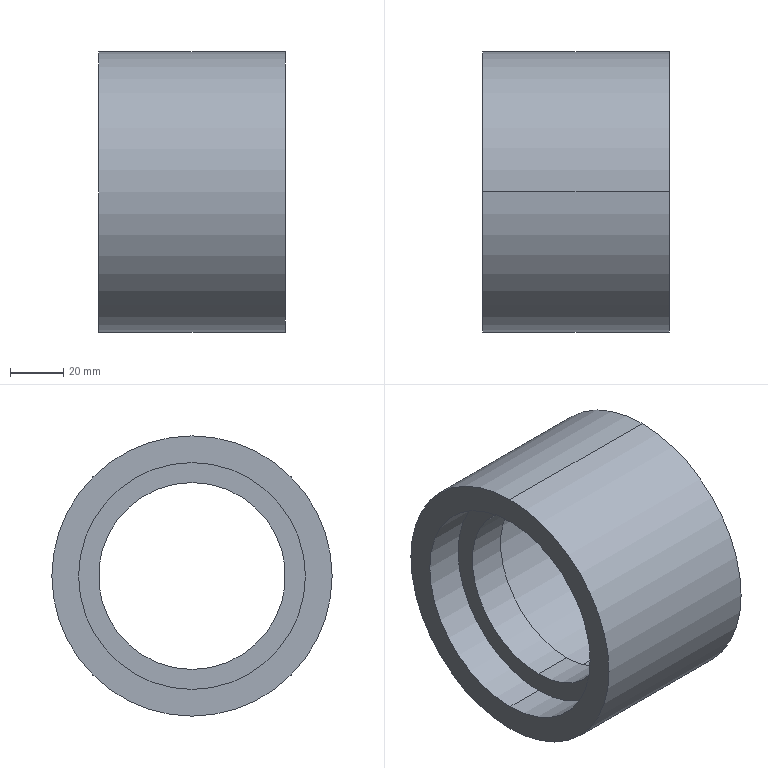Component | SolidWorks | bearing dan rumahan assembly-1_rumah bearing-1 | 1 solid | 24 faces | box 70 x 105 x 105 mm | volume 234610 mm3 | cylinder 16 | plane 8 | commonest cylinder face diameters 6 x8 85 x4 70 x2 105 x2 | material ASTM A36 Steel
build123d program:
from build123d import *

# Parameters (mm, degrees)
BOSS_EXTRUDE1_DEPTH      = 40
BOSS_EXTRUDE1_DEPTH_BACK = 30
SKETCH1_R                = 52.5
SKETCH1_R_2              = 42.5
SKETCH2_R                = 42.5
SKETCH2_R_2              = 35
BOSS_EXTRUDE2_DEPTH      = 15
SKETCH3_R                = 3
CUT_EXTRUDE1_DEPTH       = 15


with BuildPart() as part:
    # Sketch1 → Boss-Extrude1 (new, two sides: drawn at the far end of the back side and taken through both)
    with BuildSketch(Plane(origin=(0, 0, 0), x_dir=(0, 0, -1), z_dir=(1, 0, 0)).offset(-BOSS_EXTRUDE1_DEPTH_BACK)):
        Circle(SKETCH1_R)
        Circle(SKETCH1_R_2, mode=Mode.SUBTRACT)
    extrude(amount=BOSS_EXTRUDE1_DEPTH + BOSS_EXTRUDE1_DEPTH_BACK)

    # Sketch2 → Boss-Extrude2 (add)
    with BuildSketch(Plane(origin=(0, 0, 0), x_dir=(0, 0, -1), z_dir=(1, 0, 0))):
        Circle(SKETCH2_R)
        Circle(SKETCH2_R_2, mode=Mode.SUBTRACT)
    extrude(amount=-BOSS_EXTRUDE2_DEPTH)

    # Sketch3 → Cut-Extrude1 (cut)
    with BuildSketch(Plane(origin=(40, 0, 0), x_dir=(0, 0, -1), z_dir=(1, 0, 0))):
        with Locations((0, 47.5)):
            Circle(SKETCH3_R)
        with Locations((47.5, 0)):
            Circle(SKETCH3_R)
        with Locations((0, -47.5)):
            Circle(SKETCH3_R)
        with Locations((-47.5, 0)):
            Circle(SKETCH3_R)
    extrude(amount=-CUT_EXTRUDE1_DEPTH, mode=Mode.SUBTRACT)


solid = part.part

# Placed as in the assembly
solid = solid.moved(Location((-2.5, -110, 40), (0, 0, 0)))
STEP:
#1=COLOUR_RGB('',0.7922,0.8196,0.9333);
#2=FILL_AREA_STYLE_COLOUR('',#1);
#3=FILL_AREA_STYLE('',(#2));
#4=SURFACE_STYLE_FILL_AREA(#3);
#5=SURFACE_SIDE_STYLE('',(#4));
#6=SURFACE_STYLE_USAGE(.BOTH.,#5);
#7=PRESENTATION_STYLE_ASSIGNMENT((#6));
#8=CARTESIAN_POINT('',(0.8858,-2.461,1.693));
#9=VERTEX_POINT('',#8);
#10=CARTESIAN_POINT('',(0.8858,-2.461,1.457));
#11=VERTEX_POINT('',#10);
#12=CARTESIAN_POINT('',(0.8858,-2.461,1.575));
#13=DIRECTION('',(1.,-0.,-0.));
#14=DIRECTION('',(0.,0.,-1.));
#15=AXIS2_PLACEMENT_3D('',#12,#13,#14);
#16=CIRCLE('',#15,0.1181);
#17=EDGE_CURVE('',#9,#11,#16,.T.);
#18=ORIENTED_EDGE('',*,*,#17,.F.);
#19=CARTESIAN_POINT('',(1.476,-2.461,1.693));
#20=VERTEX_POINT('',#19);
#21=CARTESIAN_POINT('',(0.8858,-2.461,1.693));
#22=DIRECTION('',(1.,-0.,-0.));
#23=VECTOR('',#22,39.37);
#24=LINE('',#21,#23);
#25=EDGE_CURVE('',#9,#20,#24,.T.);
#26=ORIENTED_EDGE('',*,*,#25,.T.);
#27=CARTESIAN_POINT('',(1.476,-2.461,1.457));
#28=VERTEX_POINT('',#27);
#29=CARTESIAN_POINT('',(1.476,-2.461,1.575));
#30=DIRECTION('',(1.,-0.,-0.));
#31=DIRECTION('',(0.,0.,-1.));
#32=AXIS2_PLACEMENT_3D('',#29,#30,#31);
#33=CIRCLE('',#32,0.1181);
#34=EDGE_CURVE('',#20,#28,#33,.T.);
#35=ORIENTED_EDGE('',*,*,#34,.T.);
#36=CARTESIAN_POINT('',(0.8858,-2.461,1.457));
#37=DIRECTION('',(1.,-0.,-0.));
#38=VECTOR('',#37,39.37);
#39=LINE('',#36,#38);
#40=EDGE_CURVE('',#11,#28,#39,.T.);
#41=ORIENTED_EDGE('',*,*,#40,.F.);
#42=EDGE_LOOP('',(#18,#26,#35,#41));
#43=FACE_OUTER_BOUND('',#42,.T.);
#44=CARTESIAN_POINT('',(0.8858,-2.461,1.575));
#45=DIRECTION('',(1.,-0.,-0.));
#46=DIRECTION('',(0.,0.,-1.));
#47=AXIS2_PLACEMENT_3D('',#44,#45,#46);
#48=CYLINDRICAL_SURFACE('',#47,0.1181);
#49=ADVANCED_FACE('',(#43),#48,.F.);
#50=CARTESIAN_POINT('',(0.8858,-4.331,-0.1772));
#51=VERTEX_POINT('',#50);
#52=CARTESIAN_POINT('',(0.8858,-4.331,-0.4134));
#53=VERTEX_POINT('',#52);
#54=CARTESIAN_POINT('',(0.8858,-4.331,-0.2953));
#55=DIRECTION('',(1.,-0.,-0.));
#56=DIRECTION('',(0.,0.,-1.));
#57=AXIS2_PLACEMENT_3D('',#54,#55,#56);
#58=CIRCLE('',#57,0.1181);
#59=EDGE_CURVE('',#51,#53,#58,.T.);
#60=ORIENTED_EDGE('',*,*,#59,.F.);
#61=CARTESIAN_POINT('',(1.476,-4.331,-0.1772));
#62=VERTEX_POINT('',#61);
#63=CARTESIAN_POINT('',(0.8858,-4.331,-0.1772));
#64=DIRECTION('',(1.,-0.,-0.));
#65=VECTOR('',#64,39.37);
#66=LINE('',#63,#65);
#67=EDGE_CURVE('',#51,#62,#66,.T.);
#68=ORIENTED_EDGE('',*,*,#67,.T.);
#69=CARTESIAN_POINT('',(1.476,-4.331,-0.4134));
#70=VERTEX_POINT('',#69);
#71=CARTESIAN_POINT('',(1.476,-4.331,-0.2953));
#72=DIRECTION('',(1.,-0.,-0.));
#73=DIRECTION('',(0.,0.,-1.));
#74=AXIS2_PLACEMENT_3D('',#71,#72,#73);
#75=CIRCLE('',#74,0.1181);
#76=EDGE_CURVE('',#62,#70,#75,.T.);
#77=ORIENTED_EDGE('',*,*,#76,.T.);
#78=CARTESIAN_POINT('',(0.8858,-4.331,-0.4134));
#79=DIRECTION('',(1.,-0.,-0.));
#80=VECTOR('',#79,39.37);
#81=LINE('',#78,#80);
#82=EDGE_CURVE('',#53,#70,#81,.T.);
#83=ORIENTED_EDGE('',*,*,#82,.F.);
#84=EDGE_LOOP('',(#60,#68,#77,#83));
#85=FACE_OUTER_BOUND('',#84,.T.);
#86=CARTESIAN_POINT('',(0.8858,-4.331,-0.2953));
#87=DIRECTION('',(1.,-0.,-0.));
#88=DIRECTION('',(0.,0.,-1.));
#89=AXIS2_PLACEMENT_3D('',#86,#87,#88);
#90=CYLINDRICAL_SURFACE('',#89,0.1181);
#91=ADVANCED_FACE('',(#85),#90,.F.);
#92=CARTESIAN_POINT('',(0.8858,-6.201,1.693));
#93=VERTEX_POINT('',#92);
#94=CARTESIAN_POINT('',(0.8858,-6.201,1.457));
#95=VERTEX_POINT('',#94);
#96=CARTESIAN_POINT('',(0.8858,-6.201,1.575));
#97=DIRECTION('',(1.,-0.,-0.));
#98=DIRECTION('',(0.,0.,-1.));
#99=AXIS2_PLACEMENT_3D('',#96,#97,#98);
#100=CIRCLE('',#99,0.1181);
#101=EDGE_CURVE('',#93,#95,#100,.T.);
#102=ORIENTED_EDGE('',*,*,#101,.F.);
#103=CARTESIAN_POINT('',(1.476,-6.201,1.693));
#104=VERTEX_POINT('',#103);
#105=CARTESIAN_POINT('',(0.8858,-6.201,1.693));
#106=DIRECTION('',(1.,-0.,-0.));
#107=VECTOR('',#106,39.37);
#108=LINE('',#105,#107);
#109=EDGE_CURVE('',#93,#104,#108,.T.);
#110=ORIENTED_EDGE('',*,*,#109,.T.);
#111=CARTESIAN_POINT('',(1.476,-6.201,1.457));
#112=VERTEX_POINT('',#111);
#113=CARTESIAN_POINT('',(1.476,-6.201,1.575));
#114=DIRECTION('',(1.,-0.,-0.));
#115=DIRECTION('',(0.,0.,-1.));
#116=AXIS2_PLACEMENT_3D('',#113,#114,#115);
#117=CIRCLE('',#116,0.1181);
#118=EDGE_CURVE('',#104,#112,#117,.T.);
#119=ORIENTED_EDGE('',*,*,#118,.T.);
#120=CARTESIAN_POINT('',(0.8858,-6.201,1.457));
#121=DIRECTION('',(1.,-0.,-0.));
#122=VECTOR('',#121,39.37);
#123=LINE('',#120,#122);
#124=EDGE_CURVE('',#95,#112,#123,.T.);
#125=ORIENTED_EDGE('',*,*,#124,.F.);
#126=EDGE_LOOP('',(#102,#110,#119,#125));
#127=FACE_OUTER_BOUND('',#126,.T.);
#128=CARTESIAN_POINT('',(0.8858,-6.201,1.575));
#129=DIRECTION('',(1.,-0.,-0.));
#130=DIRECTION('',(0.,0.,-1.));
#131=AXIS2_PLACEMENT_3D('',#128,#129,#130);
#132=CYLINDRICAL_SURFACE('',#131,0.1181);
#133=ADVANCED_FACE('',(#127),#132,.F.);
#134=CARTESIAN_POINT('',(0.8858,-4.331,3.563));
#135=VERTEX_POINT('',#134);
#136=CARTESIAN_POINT('',(0.8858,-4.331,3.327));
#137=VERTEX_POINT('',#136);
#138=CARTESIAN_POINT('',(0.8858,-4.331,3.445));
#139=DIRECTION('',(1.,-0.,-0.));
#140=DIRECTION('',(0.,0.,-1.));
#141=AXIS2_PLACEMENT_3D('',#138,#139,#140);
#142=CIRCLE('',#141,0.1181);
#143=EDGE_CURVE('',#135,#137,#142,.T.);
#144=ORIENTED_EDGE('',*,*,#143,.F.);
#145=CARTESIAN_POINT('',(1.476,-4.331,3.563));
#146=VERTEX_POINT('',#145);
#147=CARTESIAN_POINT('',(0.8858,-4.331,3.563));
#148=DIRECTION('',(1.,-0.,-0.));
#149=VECTOR('',#148,39.37);
#150=LINE('',#147,#149);
#151=EDGE_CURVE('',#135,#146,#150,.T.);
#152=ORIENTED_EDGE('',*,*,#151,.T.);
#153=CARTESIAN_POINT('',(1.476,-4.331,3.327));
#154=VERTEX_POINT('',#153);
#155=CARTESIAN_POINT('',(1.476,-4.331,3.445));
#156=DIRECTION('',(1.,-0.,-0.));
#157=DIRECTION('',(0.,0.,-1.));
#158=AXIS2_PLACEMENT_3D('',#155,#156,#157);
#159=CIRCLE('',#158,0.1181);
#160=EDGE_CURVE('',#146,#154,#159,.T.);
#161=ORIENTED_EDGE('',*,*,#160,.T.);
#162=CARTESIAN_POINT('',(0.8858,-4.331,3.327));
#163=DIRECTION('',(1.,-0.,-0.));
#164=VECTOR('',#163,39.37);
#165=LINE('',#162,#164);
#166=EDGE_CURVE('',#137,#154,#165,.T.);
#167=ORIENTED_EDGE('',*,*,#166,.F.);
#168=EDGE_LOOP('',(#144,#152,#161,#167));
#169=FACE_OUTER_BOUND('',#168,.T.);
#170=CARTESIAN_POINT('',(0.8858,-4.331,3.445));
#171=DIRECTION('',(1.,-0.,-0.));
#172=DIRECTION('',(0.,0.,-1.));
#173=AXIS2_PLACEMENT_3D('',#170,#171,#172);
#174=CYLINDRICAL_SURFACE('',#173,0.1181);
#175=ADVANCED_FACE('',(#169),#174,.F.);
#176=CARTESIAN_POINT('',(-0.689,-4.331,2.953));
#177=VERTEX_POINT('',#176);
#178=CARTESIAN_POINT('',(-0.689,-4.331,0.1969));
#179=VERTEX_POINT('',#178);
#180=CARTESIAN_POINT('',(-0.689,-4.331,1.575));
#181=DIRECTION('',(1.,-0.,-0.));
#182=DIRECTION('',(-0.,0.,-1.));
#183=AXIS2_PLACEMENT_3D('',#180,#181,#182);
#184=CIRCLE('',#183,1.378);
#185=EDGE_CURVE('',#177,#179,#184,.T.);
#186=ORIENTED_EDGE('',*,*,#185,.F.);
#187=CARTESIAN_POINT('',(-0.09843,-4.331,2.953));
#188=VERTEX_POINT('',#187);
#189=CARTESIAN_POINT('',(-0.689,-4.331,2.953));
#190=DIRECTION('',(1.,-0.,-0.));
#191=VECTOR('',#190,39.37);
#192=LINE('',#189,#191);
#193=EDGE_CURVE('',#177,#188,#192,.T.);
#194=ORIENTED_EDGE('',*,*,#193,.T.);
#195=CARTESIAN_POINT('',(-0.09843,-4.331,0.1969));
#196=VERTEX_POINT('',#195);
#197=CARTESIAN_POINT('',(-0.09843,-4.331,1.575));
#198=DIRECTION('',(1.,-0.,-0.));
#199=DIRECTION('',(-0.,0.,-1.));
#200=AXIS2_PLACEMENT_3D('',#197,#198,#199);
#201=CIRCLE('',#200,1.378);
#202=EDGE_CURVE('',#188,#196,#201,.T.);
#203=ORIENTED_EDGE('',*,*,#202,.T.);
#204=CARTESIAN_POINT('',(-0.689,-4.331,0.1969));
#205=DIRECTION('',(1.,-0.,-0.));
#206=VECTOR('',#205,39.37);
#207=LINE('',#204,#206);
#208=EDGE_CURVE('',#179,#196,#207,.T.);
#209=ORIENTED_EDGE('',*,*,#208,.F.);
#210=EDGE_LOOP('',(#186,#194,#203,#209));
#211=FACE_OUTER_BOUND('',#210,.T.);
#212=CARTESIAN_POINT('',(-0.689,-4.331,1.575));
#213=DIRECTION('',(1.,-0.,-0.));
#214=DIRECTION('',(-0.,0.,-1.));
#215=AXIS2_PLACEMENT_3D('',#212,#213,#214);
#216=CYLINDRICAL_SURFACE('',#215,1.378);
#217=ADVANCED_FACE('',(#211),#216,.F.);
#218=CARTESIAN_POINT('',(-0.09843,-4.331,3.248));
#219=VERTEX_POINT('',#218);
#220=CARTESIAN_POINT('',(-0.09843,-4.331,-0.09843));
#221=VERTEX_POINT('',#220);
#222=CARTESIAN_POINT('',(-0.09843,-4.331,1.575));
#223=DIRECTION('',(1.,-0.,-0.));
#224=DIRECTION('',(-0.,0.,-1.));
#225=AXIS2_PLACEMENT_3D('',#222,#223,#224);
#226=CIRCLE('',#225,1.673);
#227=EDGE_CURVE('',#219,#221,#226,.T.);
#228=ORIENTED_EDGE('',*,*,#227,.F.);
#229=CARTESIAN_POINT('',(1.476,-4.331,3.248));
#230=VERTEX_POINT('',#229);
#231=CARTESIAN_POINT('',(-1.28,-4.331,3.248));
#232=DIRECTION('',(1.,-0.,-0.));
#233=VECTOR('',#232,39.37);
#234=LINE('',#231,#233);
#235=EDGE_CURVE('',#219,#230,#234,.T.);
#236=ORIENTED_EDGE('',*,*,#235,.T.);
#237=CARTESIAN_POINT('',(1.476,-4.331,-0.09843));
#238=VERTEX_POINT('',#237);
#239=CARTESIAN_POINT('',(1.476,-4.331,1.575));
#240=DIRECTION('',(1.,-0.,-0.));
#241=DIRECTION('',(-0.,0.,-1.));
#242=AXIS2_PLACEMENT_3D('',#239,#240,#241);
#243=CIRCLE('',#242,1.673);
#244=EDGE_CURVE('',#230,#238,#243,.T.);
#245=ORIENTED_EDGE('',*,*,#244,.T.);
#246=CARTESIAN_POINT('',(-1.28,-4.331,-0.09843));
#247=DIRECTION('',(1.,-0.,-0.));
#248=VECTOR('',#247,39.37);
#249=LINE('',#246,#248);
#250=EDGE_CURVE('',#221,#238,#249,.T.);
#251=ORIENTED_EDGE('',*,*,#250,.F.);
#252=EDGE_LOOP('',(#228,#236,#245,#251));
#253=FACE_OUTER_BOUND('',#252,.T.);
#254=CARTESIAN_POINT('',(-1.28,-4.331,1.575));
#255=DIRECTION('',(1.,-0.,-0.));
#256=DIRECTION('',(-0.,0.,-1.));
#257=AXIS2_PLACEMENT_3D('',#254,#255,#256);
#258=CYLINDRICAL_SURFACE('',#257,1.673);
#259=ADVANCED_FACE('',(#253),#258,.F.);
#260=CARTESIAN_POINT('',(-1.28,-4.331,-0.4921));
#261=VERTEX_POINT('',#260);
#262=CARTESIAN_POINT('',(-1.28,-4.331,3.642));
#263=VERTEX_POINT('',#262);
#264=CARTESIAN_POINT('',(-1.28,-4.331,1.575));
#265=DIRECTION('',(1.,-0.,-0.));
#266=DIRECTION('',(-0.,0.,-1.));
#267=AXIS2_PLACEMENT_3D('',#264,#265,#266);
#268=CIRCLE('',#267,2.067);
#269=EDGE_CURVE('',#261,#263,#268,.T.);
#270=ORIENTED_EDGE('',*,*,#269,.T.);
#271=CARTESIAN_POINT('',(1.476,-4.331,3.642));
#272=VERTEX_POINT('',#271);
#273=CARTESIAN_POINT('',(-1.28,-4.331,3.642));
#274=DIRECTION('',(1.,-0.,-0.));
#275=VECTOR('',#274,39.37);
#276=LINE('',#273,#275);
#277=EDGE_CURVE('',#263,#272,#276,.T.);
#278=ORIENTED_EDGE('',*,*,#277,.T.);
#279=CARTESIAN_POINT('',(1.476,-4.331,-0.4921));
#280=VERTEX_POINT('',#279);
#281=CARTESIAN_POINT('',(1.476,-4.331,1.575));
#282=DIRECTION('',(1.,-0.,-0.));
#283=DIRECTION('',(-0.,0.,-1.));
#284=AXIS2_PLACEMENT_3D('',#281,#282,#283);
#285=CIRCLE('',#284,2.067);
#286=EDGE_CURVE('',#280,#272,#285,.T.);
#287=ORIENTED_EDGE('',*,*,#286,.F.);
#288=CARTESIAN_POINT('',(-1.28,-4.331,-0.4921));
#289=DIRECTION('',(1.,-0.,-0.));
#290=VECTOR('',#289,39.37);
#291=LINE('',#288,#290);
#292=EDGE_CURVE('',#261,#280,#291,.T.);
#293=ORIENTED_EDGE('',*,*,#292,.F.);
#294=EDGE_LOOP('',(#270,#278,#287,#293));
#295=FACE_OUTER_BOUND('',#294,.T.);
#296=CARTESIAN_POINT('',(-1.28,-4.331,1.575));
#297=DIRECTION('',(1.,-0.,-0.));
#298=DIRECTION('',(-0.,0.,-1.));
#299=AXIS2_PLACEMENT_3D('',#296,#297,#298);
#300=CYLINDRICAL_SURFACE('',#299,2.067);
#301=ADVANCED_FACE('',(#295),#300,.T.);
#302=CARTESIAN_POINT('',(-1.28,-4.331,3.248));
#303=VERTEX_POINT('',#302);
#304=CARTESIAN_POINT('',(-1.28,-4.331,-0.09843));
#305=VERTEX_POINT('',#304);
#306=CARTESIAN_POINT('',(-1.28,-4.331,1.575));
#307=DIRECTION('',(1.,-0.,-0.));
#308=DIRECTION('',(-0.,0.,-1.));
#309=AXIS2_PLACEMENT_3D('',#306,#307,#308);
#310=CIRCLE('',#309,1.673);
#311=EDGE_CURVE('',#303,#305,#310,.T.);
#312=ORIENTED_EDGE('',*,*,#311,.F.);
#313=CARTESIAN_POINT('',(-0.689,-4.331,3.248));
#314=VERTEX_POINT('',#313);
#315=CARTESIAN_POINT('',(-1.28,-4.331,3.248));
#316=DIRECTION('',(1.,-0.,-0.));
#317=VECTOR('',#316,39.37);
#318=LINE('',#315,#317);
#319=EDGE_CURVE('',#303,#314,#318,.T.);
#320=ORIENTED_EDGE('',*,*,#319,.T.);
#321=CARTESIAN_POINT('',(-0.689,-4.331,-0.09843));
#322=VERTEX_POINT('',#321);
#323=CARTESIAN_POINT('',(-0.689,-4.331,1.575));
#324=DIRECTION('',(-1.,0.,0.));
#325=DIRECTION('',(-0.,0.,-1.));
#326=AXIS2_PLACEMENT_3D('',#323,#324,#325);
#327=CIRCLE('',#326,1.673);
#328=EDGE_CURVE('',#322,#314,#327,.T.);
#329=ORIENTED_EDGE('',*,*,#328,.F.);
#330=CARTESIAN_POINT('',(-1.28,-4.331,-0.09843));
#331=DIRECTION('',(1.,-0.,-0.));
#332=VECTOR('',#331,39.37);
#333=LINE('',#330,#332);
#334=EDGE_CURVE('',#305,#322,#333,.T.);
#335=ORIENTED_EDGE('',*,*,#334,.F.);
#336=EDGE_LOOP('',(#312,#320,#329,#335));
#337=FACE_OUTER_BOUND('',#336,.T.);
#338=CARTESIAN_POINT('',(-1.28,-4.331,1.575));
#339=DIRECTION('',(1.,-0.,-0.));
#340=DIRECTION('',(-0.,0.,-1.));
#341=AXIS2_PLACEMENT_3D('',#338,#339,#340);
#342=CYLINDRICAL_SURFACE('',#341,1.673);
#343=ADVANCED_FACE('',(#337),#342,.F.);
#344=ORIENTED_EDGE('',*,*,#319,.F.);
#345=CARTESIAN_POINT('',(-1.28,-4.331,1.575));
#346=DIRECTION('',(1.,-0.,-0.));
#347=DIRECTION('',(-0.,0.,-1.));
#348=AXIS2_PLACEMENT_3D('',#345,#346,#347);
#349=CIRCLE('',#348,1.673);
#350=EDGE_CURVE('',#305,#303,#349,.T.);
#351=ORIENTED_EDGE('',*,*,#350,.F.);
#352=ORIENTED_EDGE('',*,*,#334,.T.);
#353=CARTESIAN_POINT('',(-0.689,-4.331,1.575));
#354=DIRECTION('',(-1.,0.,0.));
#355=DIRECTION('',(-0.,0.,-1.));
#356=AXIS2_PLACEMENT_3D('',#353,#354,#355);
#357=CIRCLE('',#356,1.673);
#358=EDGE_CURVE('',#314,#322,#357,.T.);
#359=ORIENTED_EDGE('',*,*,#358,.F.);
#360=EDGE_LOOP('',(#344,#351,#352,#359));
#361=FACE_OUTER_BOUND('',#360,.T.);
#362=CARTESIAN_POINT('',(-1.28,-4.331,1.575));
#363=DIRECTION('',(1.,-0.,-0.));
#364=DIRECTION('',(-0.,0.,-1.));
#365=AXIS2_PLACEMENT_3D('',#362,#363,#364);
#366=CYLINDRICAL_SURFACE('',#365,1.673);
#367=ADVANCED_FACE('',(#361),#366,.F.);
#368=ORIENTED_EDGE('',*,*,#277,.F.);
#369=CARTESIAN_POINT('',(-1.28,-4.331,1.575));
#370=DIRECTION('',(1.,-0.,-0.));
#371=DIRECTION('',(-0.,0.,-1.));
#372=AXIS2_PLACEMENT_3D('',#369,#370,#371);
#373=CIRCLE('',#372,2.067);
#374=EDGE_CURVE('',#263,#261,#373,.T.);
#375=ORIENTED_EDGE('',*,*,#374,.T.);
#376=ORIENTED_EDGE('',*,*,#292,.T.);
#377=CARTESIAN_POINT('',(1.476,-4.331,1.575));
#378=DIRECTION('',(1.,-0.,-0.));
#379=DIRECTION('',(-0.,0.,-1.));
#380=AXIS2_PLACEMENT_3D('',#377,#378,#379);
#381=CIRCLE('',#380,2.067);
#382=EDGE_CURVE('',#272,#280,#381,.T.);
#383=ORIENTED_EDGE('',*,*,#382,.F.);
#384=EDGE_LOOP('',(#368,#375,#376,#383));
#385=FACE_OUTER_BOUND('',#384,.T.);
#386=CARTESIAN_POINT('',(-1.28,-4.331,1.575));
#387=DIRECTION('',(1.,-0.,-0.));
#388=DIRECTION('',(-0.,0.,-1.));
#389=AXIS2_PLACEMENT_3D('',#386,#387,#388);
#390=CYLINDRICAL_SURFACE('',#389,2.067);
#391=ADVANCED_FACE('',(#385),#390,.T.);
#392=ORIENTED_EDGE('',*,*,#350,.T.);
#393=ORIENTED_EDGE('',*,*,#311,.T.);
#394=EDGE_LOOP('',(#392,#393));
#395=FACE_BOUND('',#394,.T.);
#396=ORIENTED_EDGE('',*,*,#269,.F.);
#397=ORIENTED_EDGE('',*,*,#374,.F.);
#398=EDGE_LOOP('',(#396,#397));
#399=FACE_OUTER_BOUND('',#398,.T.);
#400=CARTESIAN_POINT('',(-1.28,-4.331,1.575));
#401=DIRECTION('',(1.,-0.,-0.));
#402=DIRECTION('',(-0.,0.,-1.));
#403=AXIS2_PLACEMENT_3D('',#400,#401,#402);
#404=PLANE('',#403);
#405=ADVANCED_FACE('',(#395,#399),#404,.F.);
#406=ORIENTED_EDGE('',*,*,#235,.F.);
#407=CARTESIAN_POINT('',(-0.09843,-4.331,1.575));
#408=DIRECTION('',(1.,-0.,-0.));
#409=DIRECTION('',(-0.,0.,-1.));
#410=AXIS2_PLACEMENT_3D('',#407,#408,#409);
#411=CIRCLE('',#410,1.673);
#412=EDGE_CURVE('',#221,#219,#411,.T.);
#413=ORIENTED_EDGE('',*,*,#412,.F.);
#414=ORIENTED_EDGE('',*,*,#250,.T.);
#415=CARTESIAN_POINT('',(1.476,-4.331,1.575));
#416=DIRECTION('',(1.,-0.,-0.));
#417=DIRECTION('',(-0.,0.,-1.));
#418=AXIS2_PLACEMENT_3D('',#415,#416,#417);
#419=CIRCLE('',#418,1.673);
#420=EDGE_CURVE('',#238,#230,#419,.T.);
#421=ORIENTED_EDGE('',*,*,#420,.T.);
#422=EDGE_LOOP('',(#406,#413,#414,#421));
#423=FACE_OUTER_BOUND('',#422,.T.);
#424=CARTESIAN_POINT('',(-1.28,-4.331,1.575));
#425=DIRECTION('',(1.,-0.,-0.));
#426=DIRECTION('',(-0.,0.,-1.));
#427=AXIS2_PLACEMENT_3D('',#424,#425,#426);
#428=CYLINDRICAL_SURFACE('',#427,1.673);
#429=ADVANCED_FACE('',(#423),#428,.F.);
#430=CARTESIAN_POINT('',(1.476,-2.461,1.575));
#431=DIRECTION('',(1.,-0.,-0.));
#432=DIRECTION('',(0.,0.,-1.));
#433=AXIS2_PLACEMENT_3D('',#430,#431,#432);
#434=CIRCLE('',#433,0.1181);
#435=EDGE_CURVE('',#28,#20,#434,.T.);
#436=ORIENTED_EDGE('',*,*,#435,.F.);
#437=ORIENTED_EDGE('',*,*,#34,.F.);
#438=EDGE_LOOP('',(#436,#437));
#439=FACE_BOUND('',#438,.T.);
#440=CARTESIAN_POINT('',(1.476,-4.331,-0.2953));
#441=DIRECTION('',(1.,-0.,-0.));
#442=DIRECTION('',(0.,0.,-1.));
#443=AXIS2_PLACEMENT_3D('',#440,#441,#442);
#444=CIRCLE('',#443,0.1181);
#445=EDGE_CURVE('',#70,#62,#444,.T.);
#446=ORIENTED_EDGE('',*,*,#445,.F.);
#447=ORIENTED_EDGE('',*,*,#76,.F.);
#448=EDGE_LOOP('',(#446,#447));
#449=FACE_BOUND('',#448,.T.);
#450=CARTESIAN_POINT('',(1.476,-6.201,1.575));
#451=DIRECTION('',(1.,-0.,-0.));
#452=DIRECTION('',(0.,0.,-1.));
#453=AXIS2_PLACEMENT_3D('',#450,#451,#452);
#454=CIRCLE('',#453,0.1181);
#455=EDGE_CURVE('',#112,#104,#454,.T.);
#456=ORIENTED_EDGE('',*,*,#455,.F.);
#457=ORIENTED_EDGE('',*,*,#118,.F.);
#458=EDGE_LOOP('',(#456,#457));
#459=FACE_BOUND('',#458,.T.);
#460=CARTESIAN_POINT('',(1.476,-4.331,3.445));
#461=DIRECTION('',(1.,-0.,-0.));
#462=DIRECTION('',(0.,0.,-1.));
#463=AXIS2_PLACEMENT_3D('',#460,#461,#462);
#464=CIRCLE('',#463,0.1181);
#465=EDGE_CURVE('',#154,#146,#464,.T.);
#466=ORIENTED_EDGE('',*,*,#465,.F.);
#467=ORIENTED_EDGE('',*,*,#160,.F.);
#468=EDGE_LOOP('',(#466,#467));
#469=FACE_BOUND('',#468,.T.);
#470=ORIENTED_EDGE('',*,*,#286,.T.);
#471=ORIENTED_EDGE('',*,*,#382,.T.);
#472=EDGE_LOOP('',(#470,#471));
#473=FACE_OUTER_BOUND('',#472,.T.);
#474=ORIENTED_EDGE('',*,*,#420,.F.);
#475=ORIENTED_EDGE('',*,*,#244,.F.);
#476=EDGE_LOOP('',(#474,#475));
#477=FACE_BOUND('',#476,.T.);
#478=CARTESIAN_POINT('',(1.476,-4.331,1.575));
#479=DIRECTION('',(1.,-0.,-0.));
#480=DIRECTION('',(-0.,0.,-1.));
#481=AXIS2_PLACEMENT_3D('',#478,#479,#480);
#482=PLANE('',#481);
#483=ADVANCED_FACE('',(#439,#449,#459,#469,#473,#477),#482,.T.);
#484=CARTESIAN_POINT('',(-0.689,-4.331,1.575));
#485=DIRECTION('',(1.,-0.,-0.));
#486=DIRECTION('',(-0.,0.,-1.));
#487=AXIS2_PLACEMENT_3D('',#484,#485,#486);
#488=CIRCLE('',#487,1.378);
#489=EDGE_CURVE('',#179,#177,#488,.T.);
#490=ORIENTED_EDGE('',*,*,#489,.T.);
#491=ORIENTED_EDGE('',*,*,#185,.T.);
#492=EDGE_LOOP('',(#490,#491));
#493=FACE_BOUND('',#492,.T.);
#494=ORIENTED_EDGE('',*,*,#328,.T.);
#495=ORIENTED_EDGE('',*,*,#358,.T.);
#496=EDGE_LOOP('',(#494,#495));
#497=FACE_OUTER_BOUND('',#496,.T.);
#498=CARTESIAN_POINT('',(-0.689,-4.331,1.575));
#499=DIRECTION('',(1.,-0.,-0.));
#500=DIRECTION('',(-0.,0.,-1.));
#501=AXIS2_PLACEMENT_3D('',#498,#499,#500);
#502=PLANE('',#501);
#503=ADVANCED_FACE('',(#493,#497),#502,.F.);
#504=CARTESIAN_POINT('',(-0.09843,-4.331,1.575));
#505=DIRECTION('',(1.,-0.,-0.));
#506=DIRECTION('',(-0.,0.,-1.));
#507=AXIS2_PLACEMENT_3D('',#504,#505,#506);
#508=CIRCLE('',#507,1.378);
#509=EDGE_CURVE('',#196,#188,#508,.T.);
#510=ORIENTED_EDGE('',*,*,#509,.F.);
#511=ORIENTED_EDGE('',*,*,#202,.F.);
#512=EDGE_LOOP('',(#510,#511));
#513=FACE_BOUND('',#512,.T.);
#514=ORIENTED_EDGE('',*,*,#412,.T.);
#515=ORIENTED_EDGE('',*,*,#227,.T.);
#516=EDGE_LOOP('',(#514,#515));
#517=FACE_OUTER_BOUND('',#516,.T.);
#518=CARTESIAN_POINT('',(-0.09843,-4.331,1.575));
#519=DIRECTION('',(1.,-0.,-0.));
#520=DIRECTION('',(-0.,0.,-1.));
#521=AXIS2_PLACEMENT_3D('',#518,#519,#520);
#522=PLANE('',#521);
#523=ADVANCED_FACE('',(#513,#517),#522,.T.);
#524=ORIENTED_EDGE('',*,*,#193,.F.);
#525=ORIENTED_EDGE('',*,*,#489,.F.);
#526=ORIENTED_EDGE('',*,*,#208,.T.);
#527=ORIENTED_EDGE('',*,*,#509,.T.);
#528=EDGE_LOOP('',(#524,#525,#526,#527));
#529=FACE_OUTER_BOUND('',#528,.T.);
#530=CARTESIAN_POINT('',(-0.689,-4.331,1.575));
#531=DIRECTION('',(1.,-0.,-0.));
#532=DIRECTION('',(-0.,0.,-1.));
#533=AXIS2_PLACEMENT_3D('',#530,#531,#532);
#534=CYLINDRICAL_SURFACE('',#533,1.378);
#535=ADVANCED_FACE('',(#529),#534,.F.);
#536=ORIENTED_EDGE('',*,*,#151,.F.);
#537=CARTESIAN_POINT('',(0.8858,-4.331,3.445));
#538=DIRECTION('',(1.,-0.,-0.));
#539=DIRECTION('',(0.,0.,-1.));
#540=AXIS2_PLACEMENT_3D('',#537,#538,#539);
#541=CIRCLE('',#540,0.1181);
#542=EDGE_CURVE('',#137,#135,#541,.T.);
#543=ORIENTED_EDGE('',*,*,#542,.F.);
#544=ORIENTED_EDGE('',*,*,#166,.T.);
#545=ORIENTED_EDGE('',*,*,#465,.T.);
#546=EDGE_LOOP('',(#536,#543,#544,#545));
#547=FACE_OUTER_BOUND('',#546,.T.);
#548=CARTESIAN_POINT('',(0.8858,-4.331,3.445));
#549=DIRECTION('',(1.,-0.,-0.));
#550=DIRECTION('',(0.,0.,-1.));
#551=AXIS2_PLACEMENT_3D('',#548,#549,#550);
#552=CYLINDRICAL_SURFACE('',#551,0.1181);
#553=ADVANCED_FACE('',(#547),#552,.F.);
#554=ORIENTED_EDGE('',*,*,#542,.T.);
#555=ORIENTED_EDGE('',*,*,#143,.T.);
#556=EDGE_LOOP('',(#554,#555));
#557=FACE_OUTER_BOUND('',#556,.T.);
#558=CARTESIAN_POINT('',(0.8858,-4.331,3.445));
#559=DIRECTION('',(1.,-0.,-0.));
#560=DIRECTION('',(-0.,0.,-1.));
#561=AXIS2_PLACEMENT_3D('',#558,#559,#560);
#562=PLANE('',#561);
#563=ADVANCED_FACE('',(#557),#562,.T.);
#564=ORIENTED_EDGE('',*,*,#109,.F.);
#565=CARTESIAN_POINT('',(0.8858,-6.201,1.575));
#566=DIRECTION('',(1.,-0.,-0.));
#567=DIRECTION('',(0.,0.,-1.));
#568=AXIS2_PLACEMENT_3D('',#565,#566,#567);
#569=CIRCLE('',#568,0.1181);
#570=EDGE_CURVE('',#95,#93,#569,.T.);
#571=ORIENTED_EDGE('',*,*,#570,.F.);
#572=ORIENTED_EDGE('',*,*,#124,.T.);
#573=ORIENTED_EDGE('',*,*,#455,.T.);
#574=EDGE_LOOP('',(#564,#571,#572,#573));
#575=FACE_OUTER_BOUND('',#574,.T.);
#576=CARTESIAN_POINT('',(0.8858,-6.201,1.575));
#577=DIRECTION('',(1.,-0.,-0.));
#578=DIRECTION('',(0.,0.,-1.));
#579=AXIS2_PLACEMENT_3D('',#576,#577,#578);
#580=CYLINDRICAL_SURFACE('',#579,0.1181);
#581=ADVANCED_FACE('',(#575),#580,.F.);
#582=ORIENTED_EDGE('',*,*,#570,.T.);
#583=ORIENTED_EDGE('',*,*,#101,.T.);
#584=EDGE_LOOP('',(#582,#583));
#585=FACE_OUTER_BOUND('',#584,.T.);
#586=CARTESIAN_POINT('',(0.8858,-6.201,1.575));
#587=DIRECTION('',(1.,-0.,-0.));
#588=DIRECTION('',(-0.,0.,-1.));
#589=AXIS2_PLACEMENT_3D('',#586,#587,#588);
#590=PLANE('',#589);
#591=ADVANCED_FACE('',(#585),#590,.T.);
#592=ORIENTED_EDGE('',*,*,#67,.F.);
#593=CARTESIAN_POINT('',(0.8858,-4.331,-0.2953));
#594=DIRECTION('',(1.,-0.,-0.));
#595=DIRECTION('',(0.,0.,-1.));
#596=AXIS2_PLACEMENT_3D('',#593,#594,#595);
#597=CIRCLE('',#596,0.1181);
#598=EDGE_CURVE('',#53,#51,#597,.T.);
#599=ORIENTED_EDGE('',*,*,#598,.F.);
#600=ORIENTED_EDGE('',*,*,#82,.T.);
#601=ORIENTED_EDGE('',*,*,#445,.T.);
#602=EDGE_LOOP('',(#592,#599,#600,#601));
#603=FACE_OUTER_BOUND('',#602,.T.);
#604=CARTESIAN_POINT('',(0.8858,-4.331,-0.2953));
#605=DIRECTION('',(1.,-0.,-0.));
#606=DIRECTION('',(0.,0.,-1.));
#607=AXIS2_PLACEMENT_3D('',#604,#605,#606);
#608=CYLINDRICAL_SURFACE('',#607,0.1181);
#609=ADVANCED_FACE('',(#603),#608,.F.);
#610=ORIENTED_EDGE('',*,*,#598,.T.);
#611=ORIENTED_EDGE('',*,*,#59,.T.);
#612=EDGE_LOOP('',(#610,#611));
#613=FACE_OUTER_BOUND('',#612,.T.);
#614=CARTESIAN_POINT('',(0.8858,-4.331,-0.2953));
#615=DIRECTION('',(1.,-0.,-0.));
#616=DIRECTION('',(-0.,0.,-1.));
#617=AXIS2_PLACEMENT_3D('',#614,#615,#616);
#618=PLANE('',#617);
#619=ADVANCED_FACE('',(#613),#618,.T.);
#620=ORIENTED_EDGE('',*,*,#25,.F.);
#621=CARTESIAN_POINT('',(0.8858,-2.461,1.575));
#622=DIRECTION('',(1.,-0.,-0.));
#623=DIRECTION('',(0.,0.,-1.));
#624=AXIS2_PLACEMENT_3D('',#621,#622,#623);
#625=CIRCLE('',#624,0.1181);
#626=EDGE_CURVE('',#11,#9,#625,.T.);
#627=ORIENTED_EDGE('',*,*,#626,.F.);
#628=ORIENTED_EDGE('',*,*,#40,.T.);
#629=ORIENTED_EDGE('',*,*,#435,.T.);
#630=EDGE_LOOP('',(#620,#627,#628,#629));
#631=FACE_OUTER_BOUND('',#630,.T.);
#632=CARTESIAN_POINT('',(0.8858,-2.461,1.575));
#633=DIRECTION('',(1.,-0.,-0.));
#634=DIRECTION('',(0.,0.,-1.));
#635=AXIS2_PLACEMENT_3D('',#632,#633,#634);
#636=CYLINDRICAL_SURFACE('',#635,0.1181);
#637=ADVANCED_FACE('',(#631),#636,.F.);
#638=ORIENTED_EDGE('',*,*,#626,.T.);
#639=ORIENTED_EDGE('',*,*,#17,.T.);
#640=EDGE_LOOP('',(#638,#639));
#641=FACE_OUTER_BOUND('',#640,.T.);
#642=CARTESIAN_POINT('',(0.8858,-2.461,1.575));
#643=DIRECTION('',(1.,-0.,-0.));
#644=DIRECTION('',(-0.,0.,-1.));
#645=AXIS2_PLACEMENT_3D('',#642,#643,#644);
#646=PLANE('',#645);
#647=ADVANCED_FACE('',(#641),#646,.T.);
#648=CLOSED_SHELL('',(#49,#91,#133,#175,#217,#259,#301,#343,#367,#391,#405,#429,#483,#503,#523,#535,#553,#563,#581,#591,#609,#619,#637,#647));
#649=MANIFOLD_SOLID_BREP('',#648);
#650=STYLED_ITEM('',(#7),#649);
#651=(LENGTH_UNIT()NAMED_UNIT(*)SI_UNIT($,.METRE.));
#652=LENGTH_MEASURE_WITH_UNIT(LENGTH_MEASURE(0.0254),#651);
#653=DIMENSIONAL_EXPONENTS(1.,0.,0.,0.,0.,0.,0.);
#654=(CONVERSION_BASED_UNIT('',#652)LENGTH_UNIT()NAMED_UNIT(#653));
#655=UNCERTAINTY_MEASURE_WITH_UNIT(LENGTH_MEASURE(0.00001),#654,'','');
#656=(NAMED_UNIT(*)PLANE_ANGLE_UNIT()SI_UNIT($,.RADIAN.));
#657=(NAMED_UNIT(*)SI_UNIT($,.STERADIAN.)SOLID_ANGLE_UNIT());
#658=(GEOMETRIC_REPRESENTATION_CONTEXT(3)GLOBAL_UNCERTAINTY_ASSIGNED_CONTEXT((#655))GLOBAL_UNIT_ASSIGNED_CONTEXT((#654,#656,#657))REPRESENTATION_CONTEXT('',''));
#659=MECHANICAL_DESIGN_GEOMETRIC_PRESENTATION_REPRESENTATION('',(#650),#658);
#660=PRESENTATION_LAYER_ASSIGNMENT('','',(#650));
#661=CARTESIAN_POINT('',(0.,0.,0.));
#662=DIRECTION('',(0.,0.,1.));
#663=DIRECTION('',(1.,0.,0.));
#664=AXIS2_PLACEMENT_3D('',#661,#662,#663);
#665=(LENGTH_UNIT()NAMED_UNIT(*)SI_UNIT($,.METRE.));
#666=LENGTH_MEASURE_WITH_UNIT(LENGTH_MEASURE(0.0254),#665);
#667=DIMENSIONAL_EXPONENTS(1.,0.,0.,0.,0.,0.,0.);
#668=(CONVERSION_BASED_UNIT('',#666)LENGTH_UNIT()NAMED_UNIT(#667));
#669=UNCERTAINTY_MEASURE_WITH_UNIT(LENGTH_MEASURE(0.00001),#668,'','');
#670=(NAMED_UNIT(*)PLANE_ANGLE_UNIT()SI_UNIT($,.RADIAN.));
#671=(NAMED_UNIT(*)SI_UNIT($,.STERADIAN.)SOLID_ANGLE_UNIT());
#672=(GEOMETRIC_REPRESENTATION_CONTEXT(3)GLOBAL_UNCERTAINTY_ASSIGNED_CONTEXT((#669))GLOBAL_UNIT_ASSIGNED_CONTEXT((#668,#670,#671))REPRESENTATION_CONTEXT('',''));
#673=ADVANCED_BREP_SHAPE_REPRESENTATION('',(#649,#664),#672);